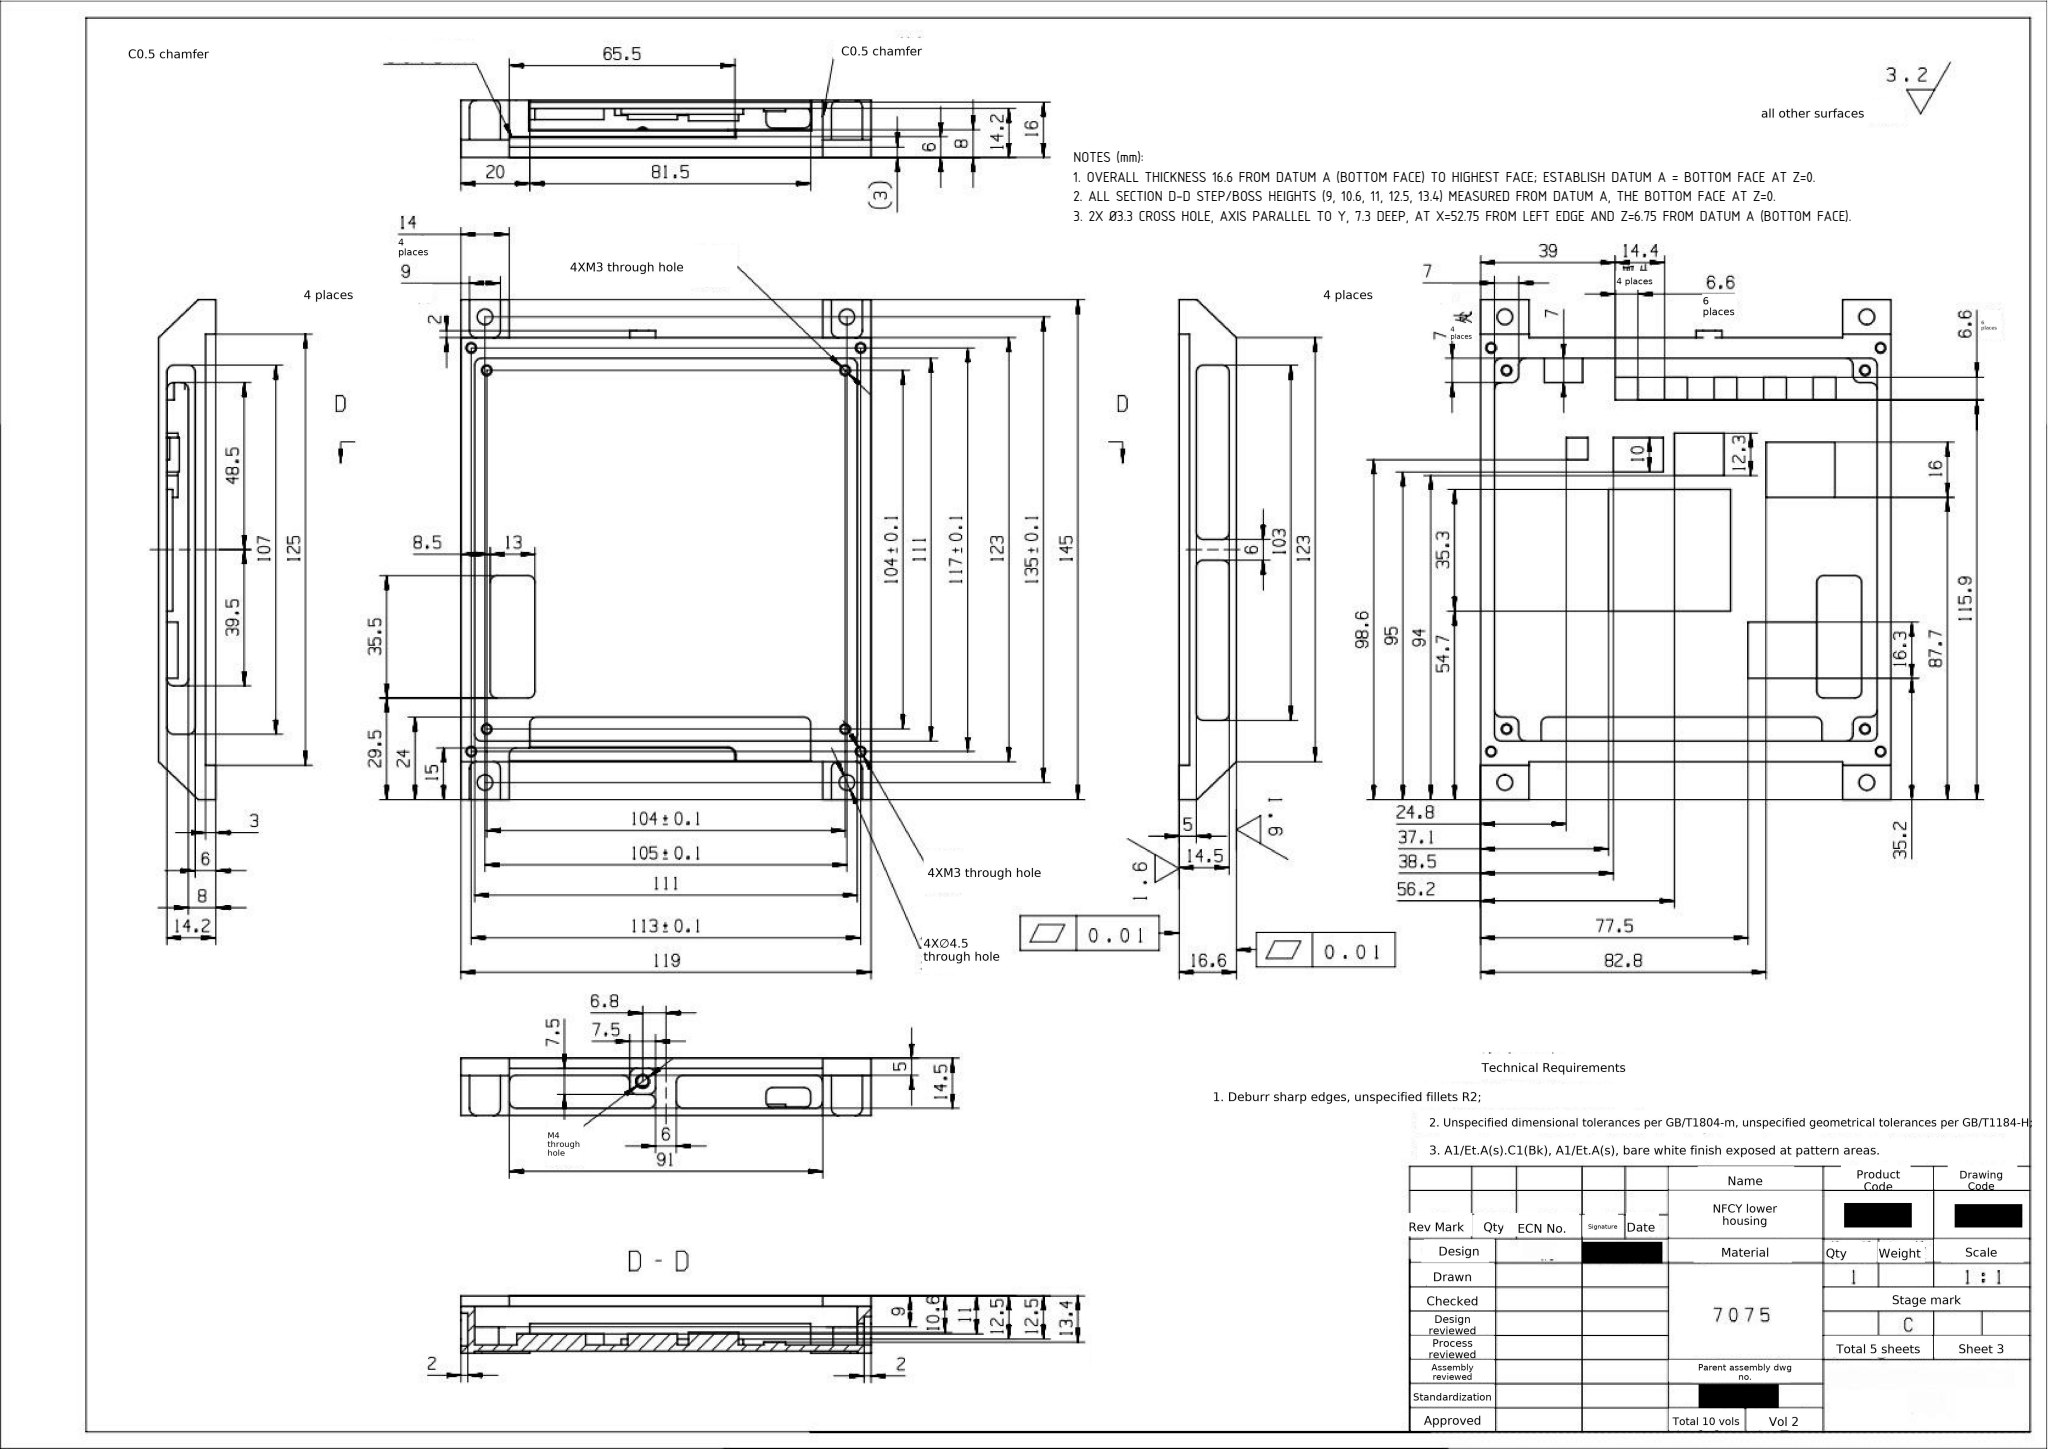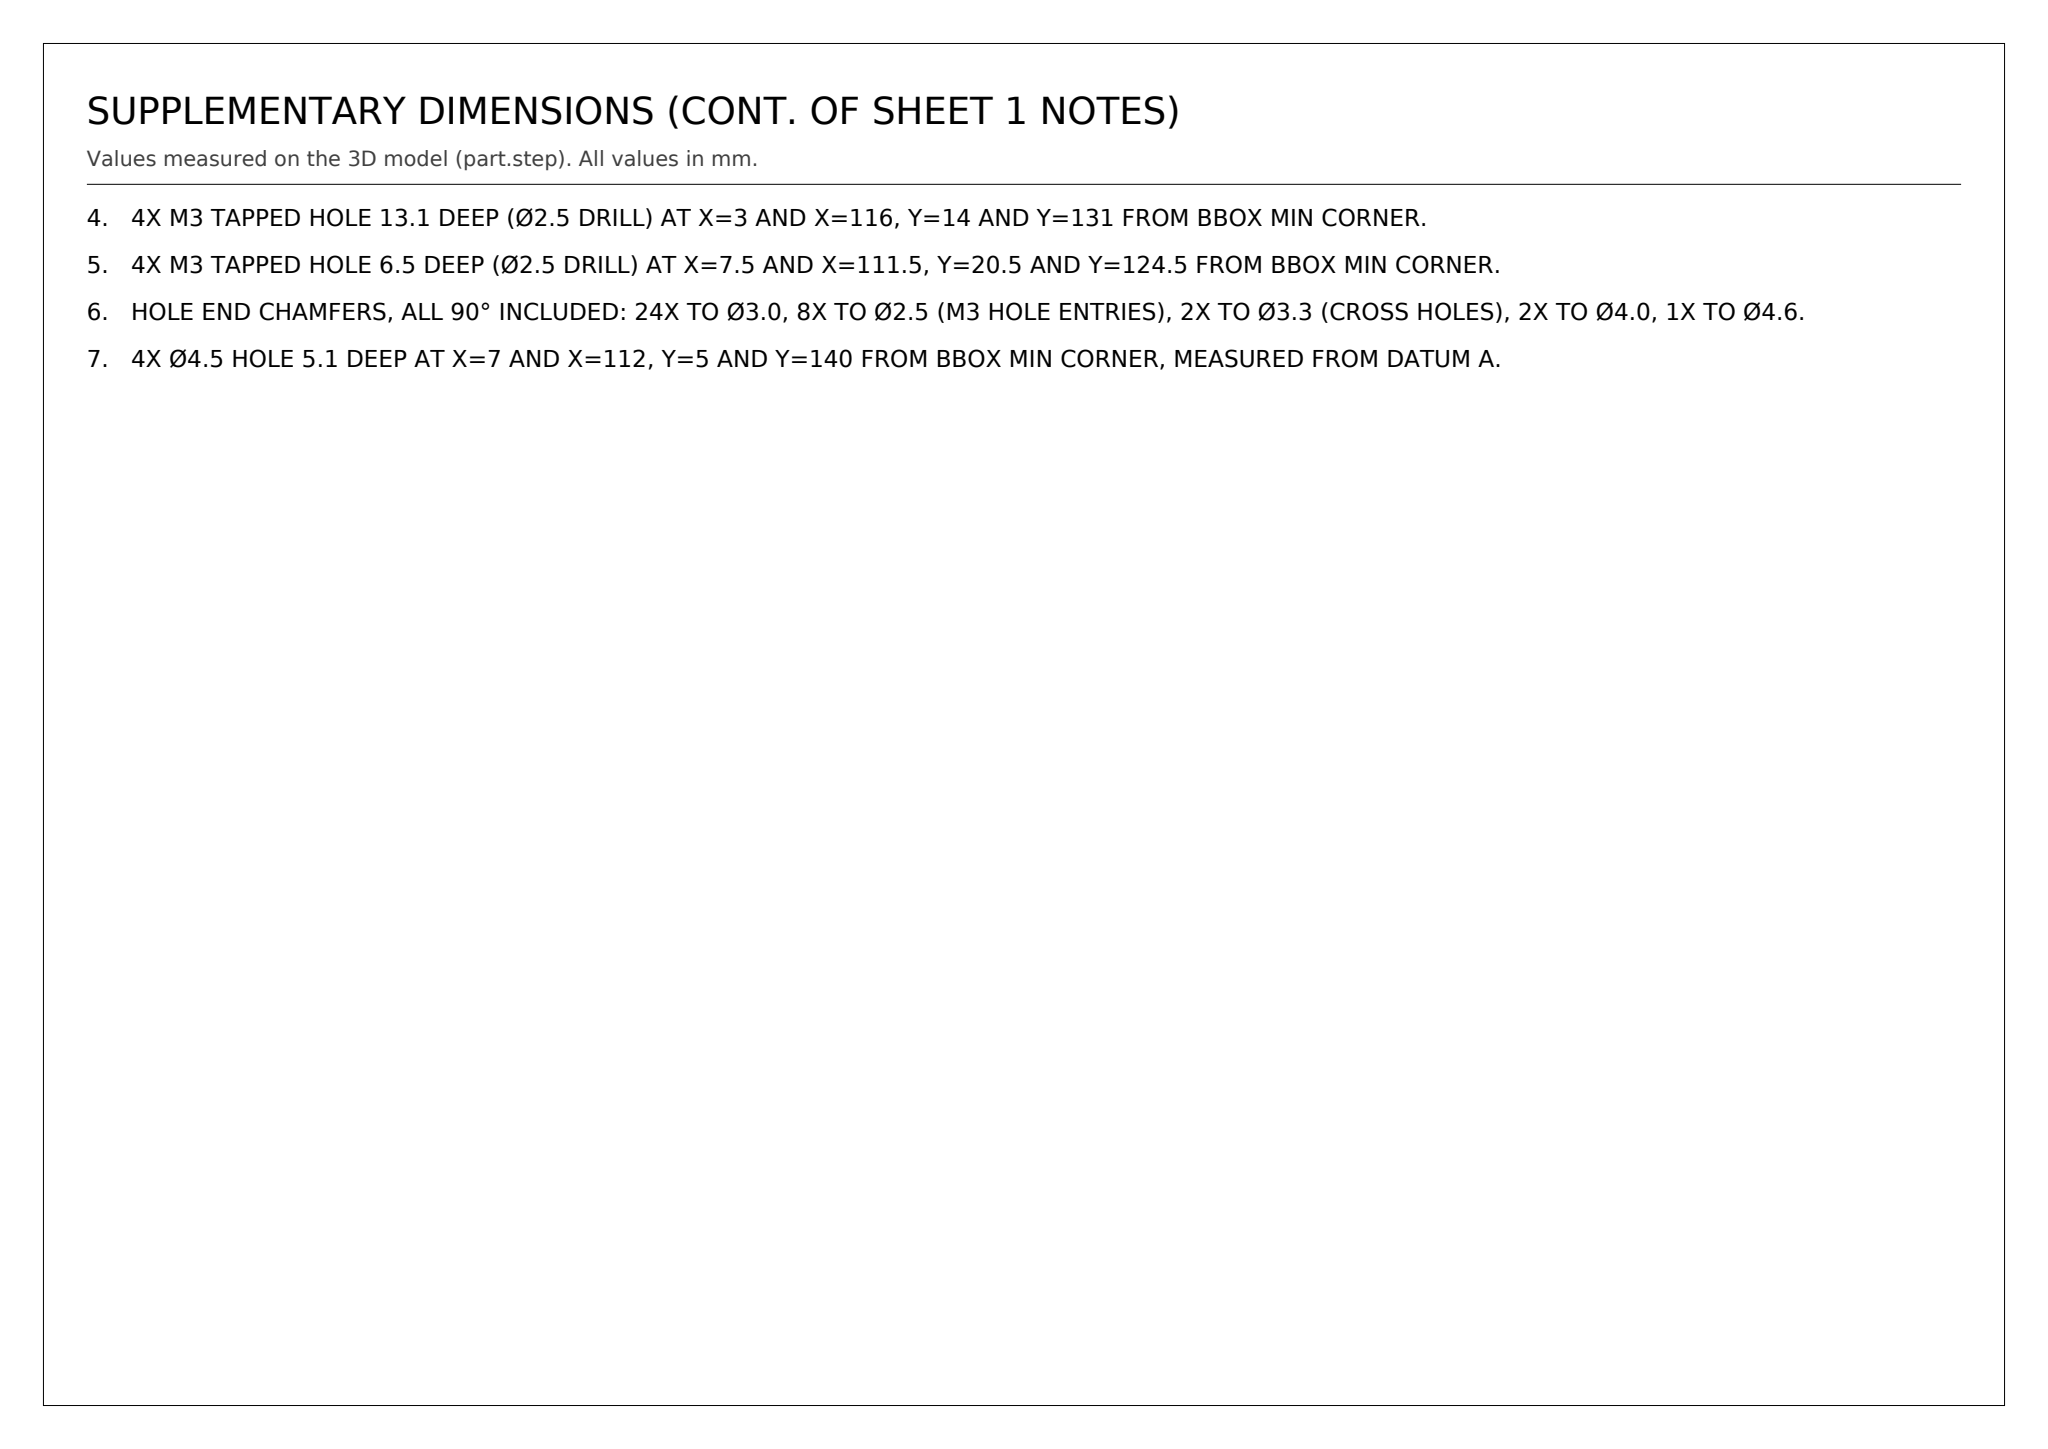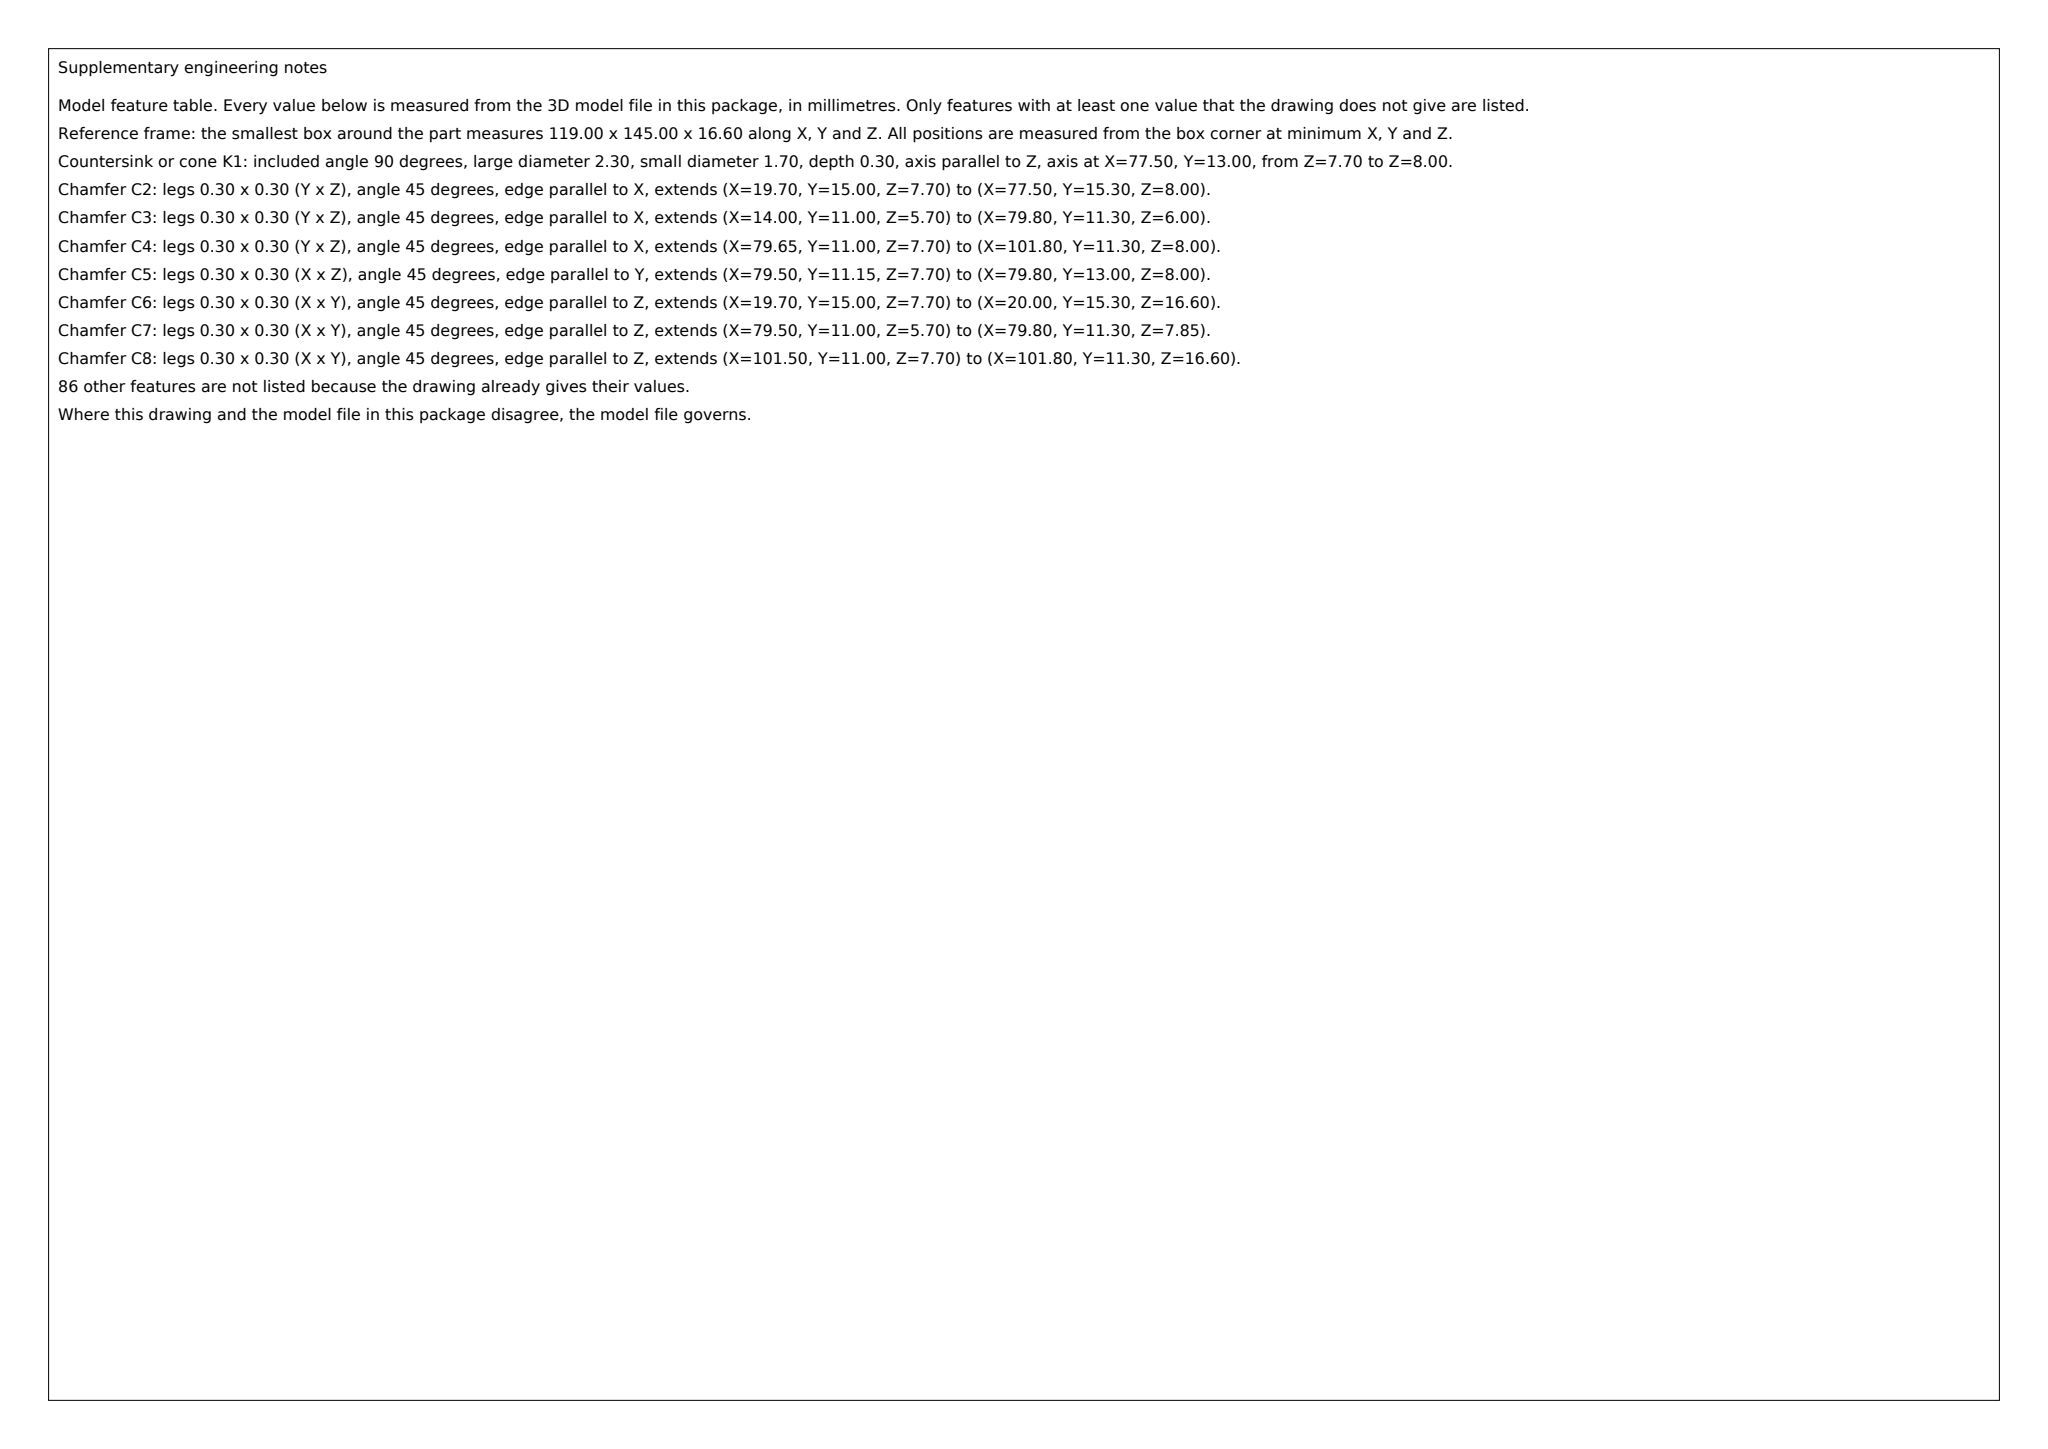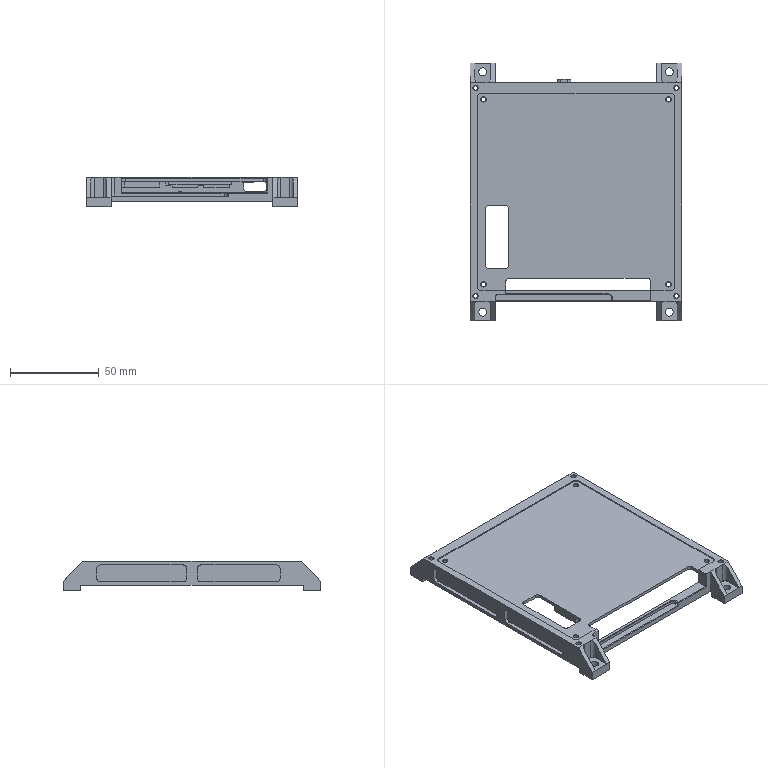Part | SolidWorks | mm | 1 solid | 304 faces | box 119 x 145 x 16.6 mm | volume 49457 mm3 | plane 173 | cylinder 94 | cone 37 | commonest cylinder face diameters 4 x68 2.5 x16 4.5 x8 3.3 x2
Drawing notes:
OVERALL THICKNESS 16.6 FROM DATUM A (BOTTOM FACE) TO HIGHEST FACE; ESTABLISH DATUM A = BOTTOM FACE AT Z=0. | from the solid: bbox_xyz z = 16.6; axis_planes ["z",0.0,4] (bottom face)
ALL SECTION D-D STEP/BOSS HEIGHTS (9, 10.6, 11, 12.5, 13.4) MEASURED FROM DATUM A, THE BOTTOM FACE AT Z=0. | from the solid: axis_planes ["z",0.0,4] single common bottom plane
2X Ø3.3 CROSS HOLE, AXIS PARALLEL TO Y, 7.3 DEEP, AT X=52.75 FROM LEFT EDGE AND Z=6.75 FROM DATUM A (BOTTOM FACE). | from the solid: cylinders [3.3,"y",[52.75,null,6.75],7.3,2]
4X M3 TAPPED HOLE 13.1 DEEP (Ø2.5 DRILL) AT X=3 AND X=116, Y=14 AND Y=131 FROM BBOX MIN CORNER. | from the solid: cylinders [2.5,"z",[3.0,14.0],13.1], [2.5,"z",[3.0,131.0],13.1], [2.5,"z",[116.0,14.0],13.1], [2.5,"z",[116.0,131.0],13.1]
4X M3 TAPPED HOLE 6.5 DEEP (Ø2.5 DRILL) AT X=7.5 AND X=111.5, Y=20.5 AND Y=124.5 FROM BBOX MIN CORNER. | from the solid: cylinders [2.5,"z",[7.5,20.5],6.5], [2.5,"z",[7.5,124.5],6.5], [2.5,"z",[111.5,20.5],6.5], [2.5,"z",[111.5,124.5],6.5]
HOLE END CHAMFERS, ALL 90° INCLUDED: 24X TO Ø3.0, 8X TO Ø2.5 (M3 HOLE ENTRIES), 2X TO Ø3.3 (CROSS HOLES), 2X TO Ø4.0, 1X TO Ø4.6. | from the solid: cones [90.0,2.5,8], [90.0,3.0,24], [90.0,3.3,2], [90.0,4.0,2], [90.0,4.6,1]
4X Ø4.5 HOLE 5.1 DEEP AT X=7 AND X=112, Y=5 AND Y=140 FROM BBOX MIN CORNER, MEASURED FROM DATUM A. | from the solid: cylinders [4.5,"z",[7.0,5.0],5.1], [4.5,"z",[7.0,140.0],5.1], [4.5,"z",[112.0,5.0],5.1]